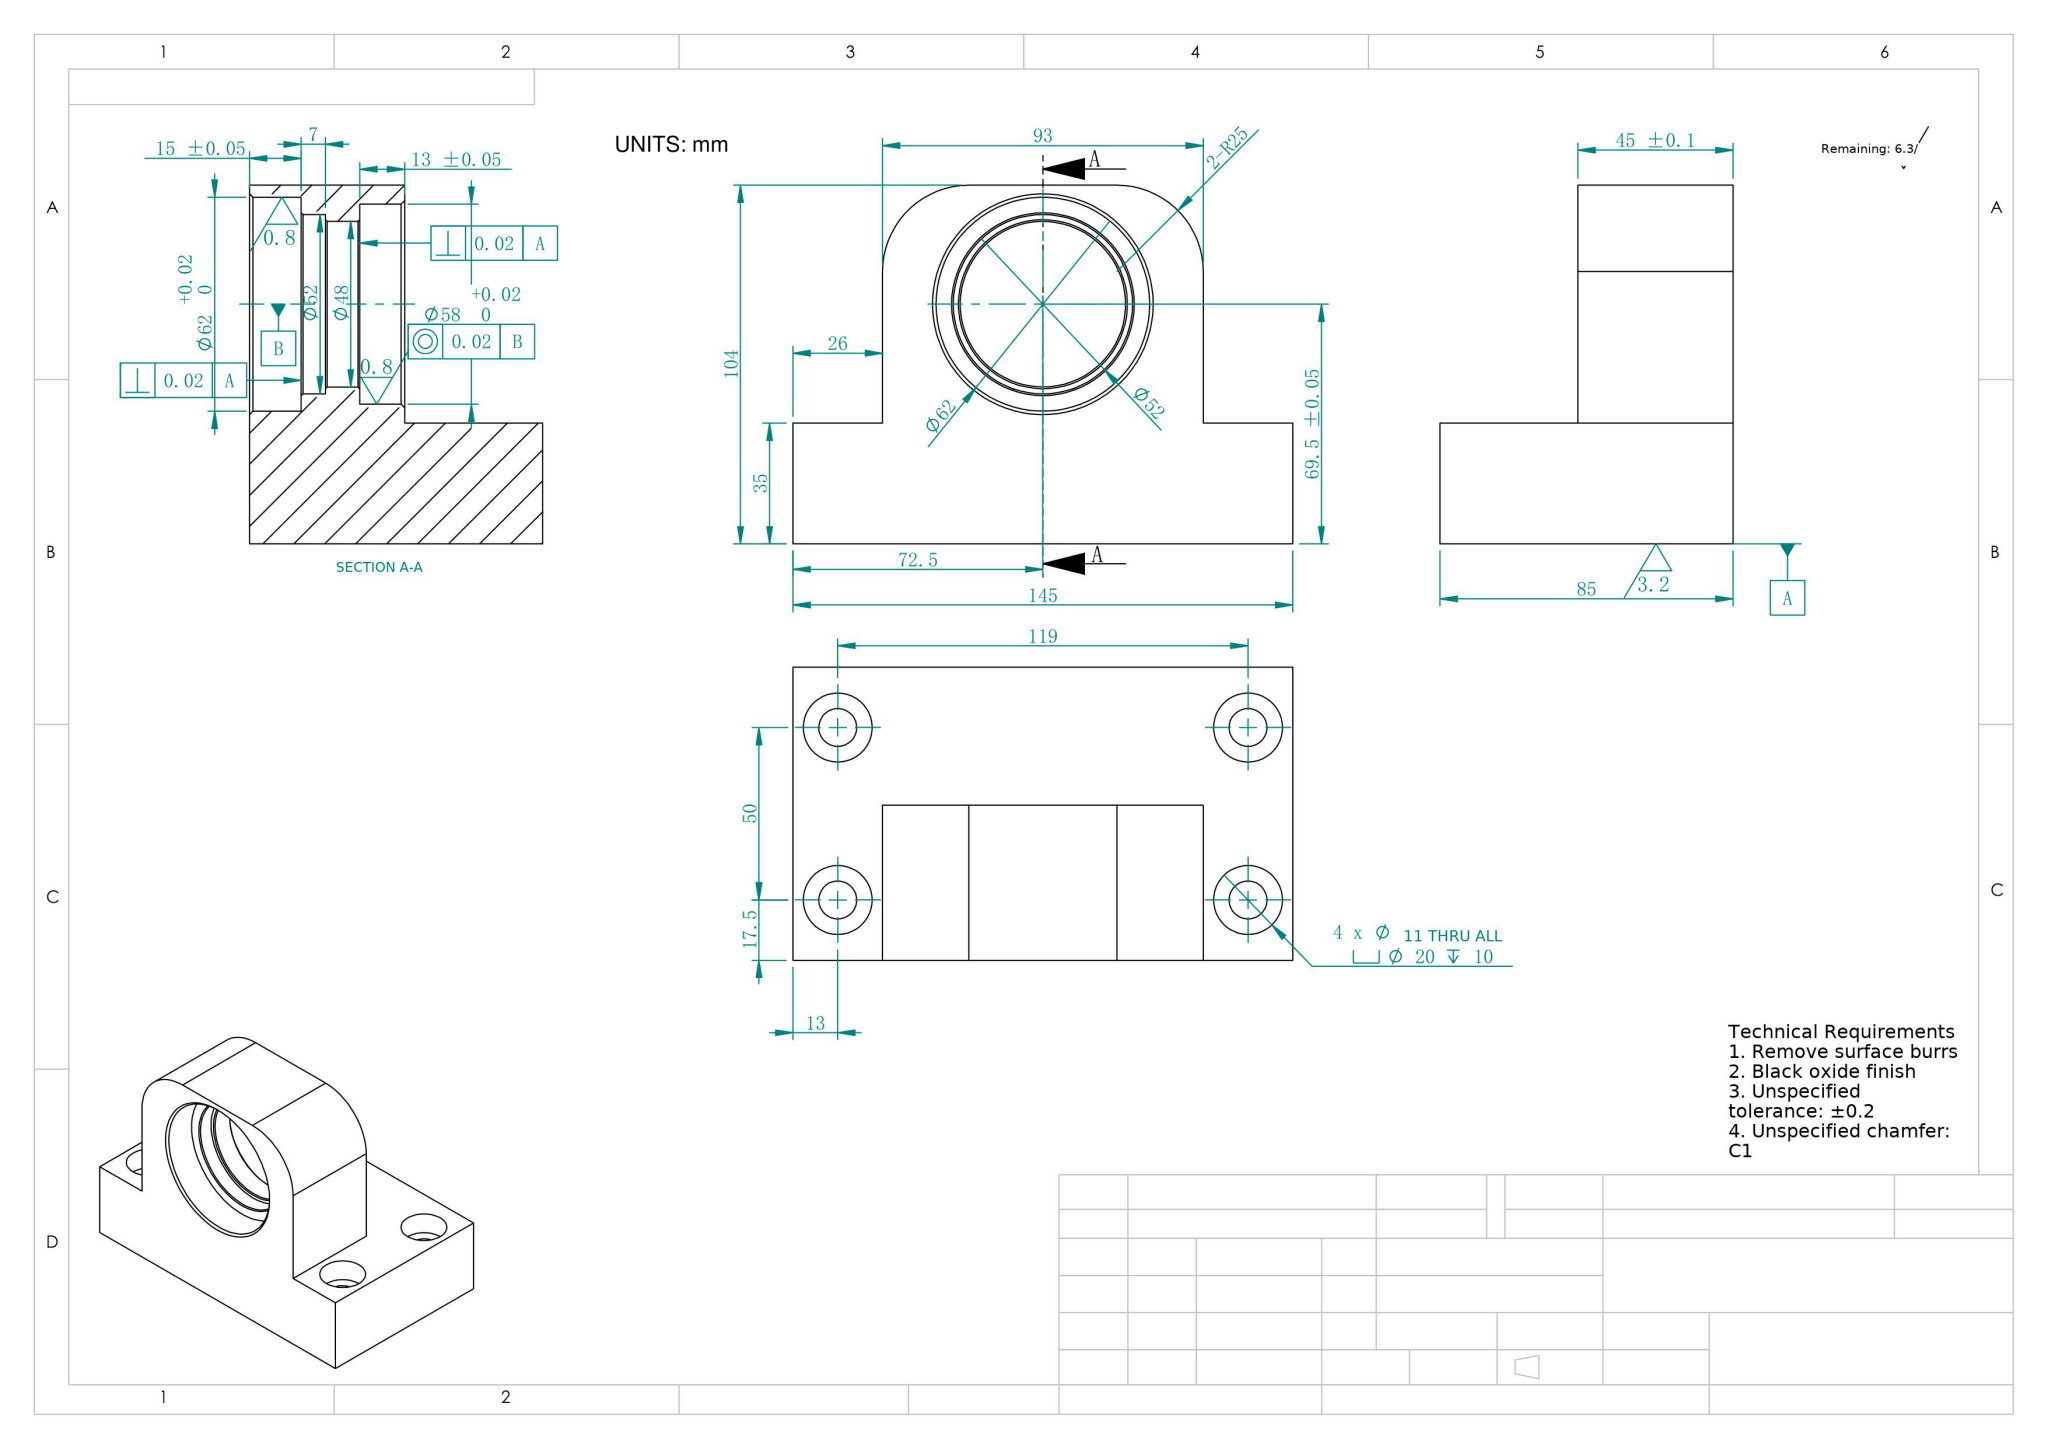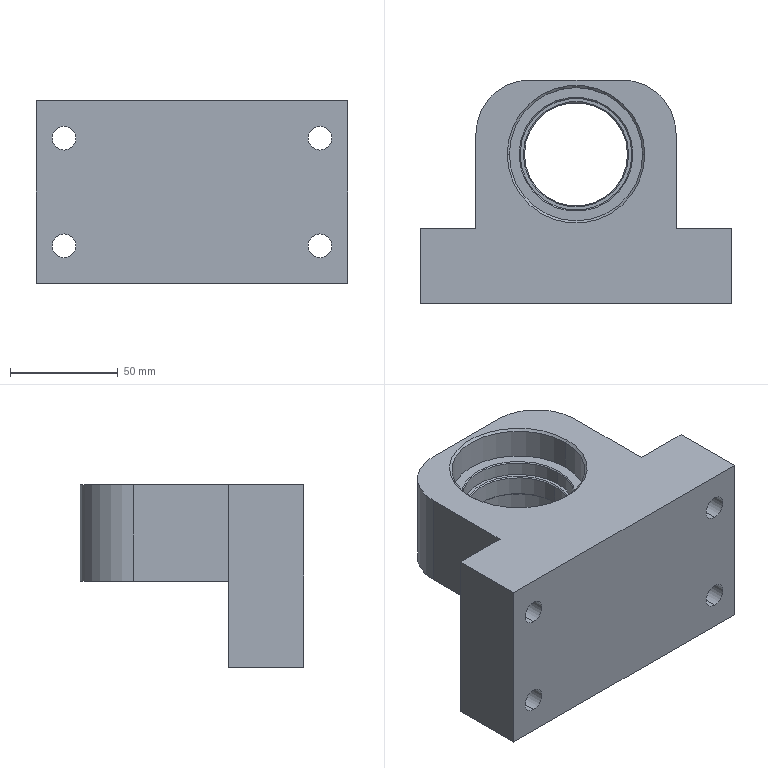Part | NX | mm | 1 solid | 53 faces | box 145 x 104 x 85 mm | volume 573155 mm3 | cylinder 26 | plane 17 | cone 10 | commonest cylinder face diameters 20 x8 11 x8 48 x2 58 x2 62 x2 52 x2 50 x2